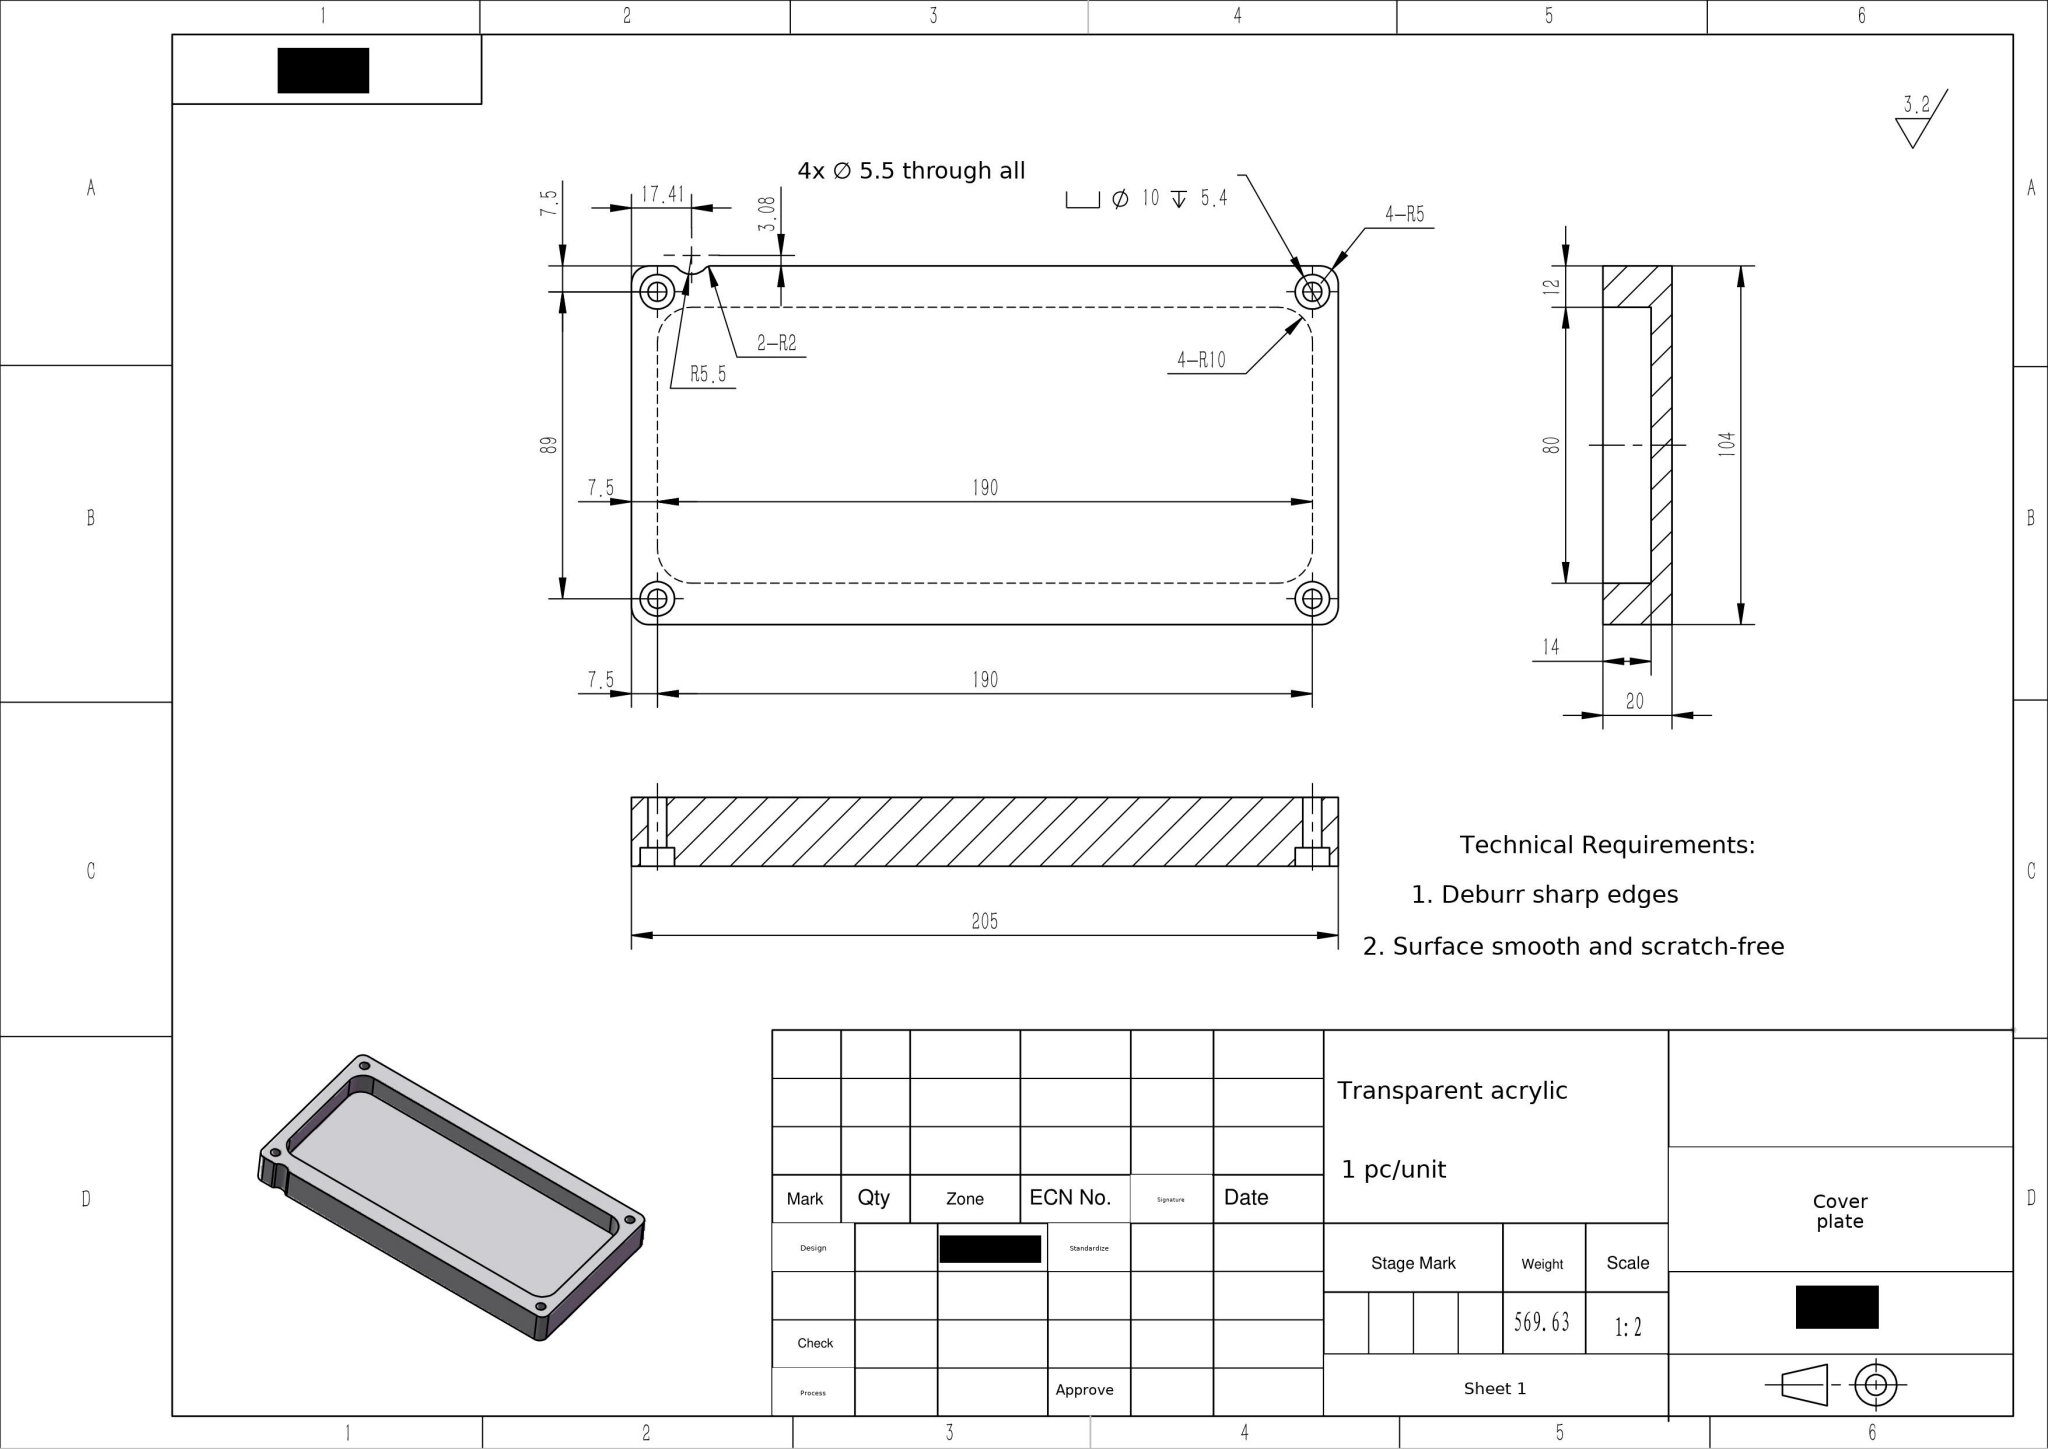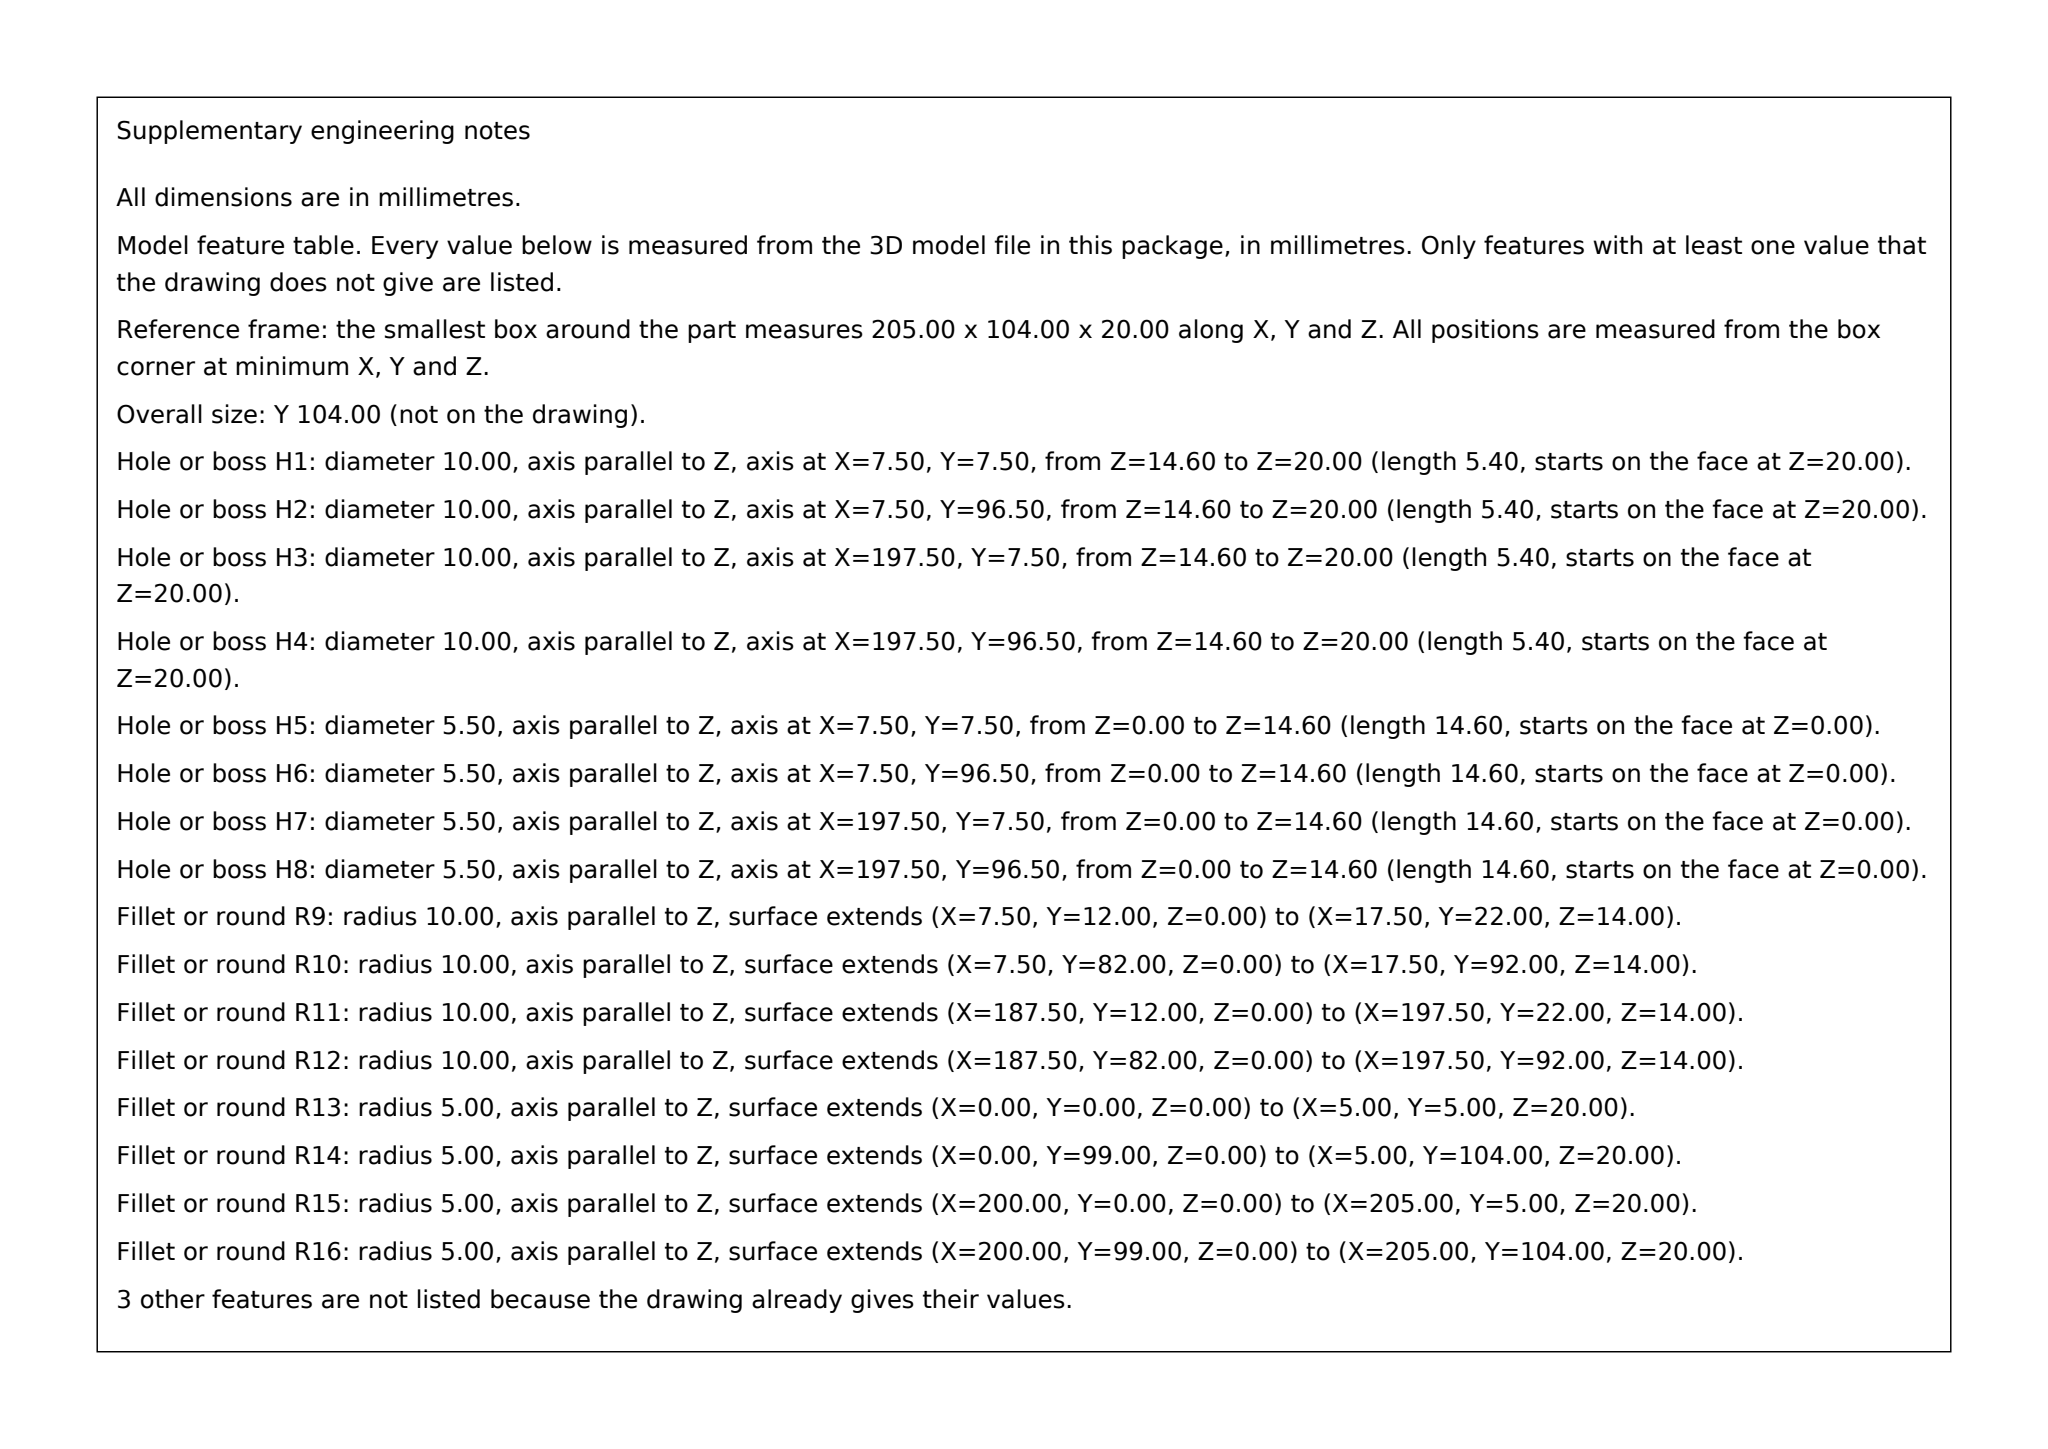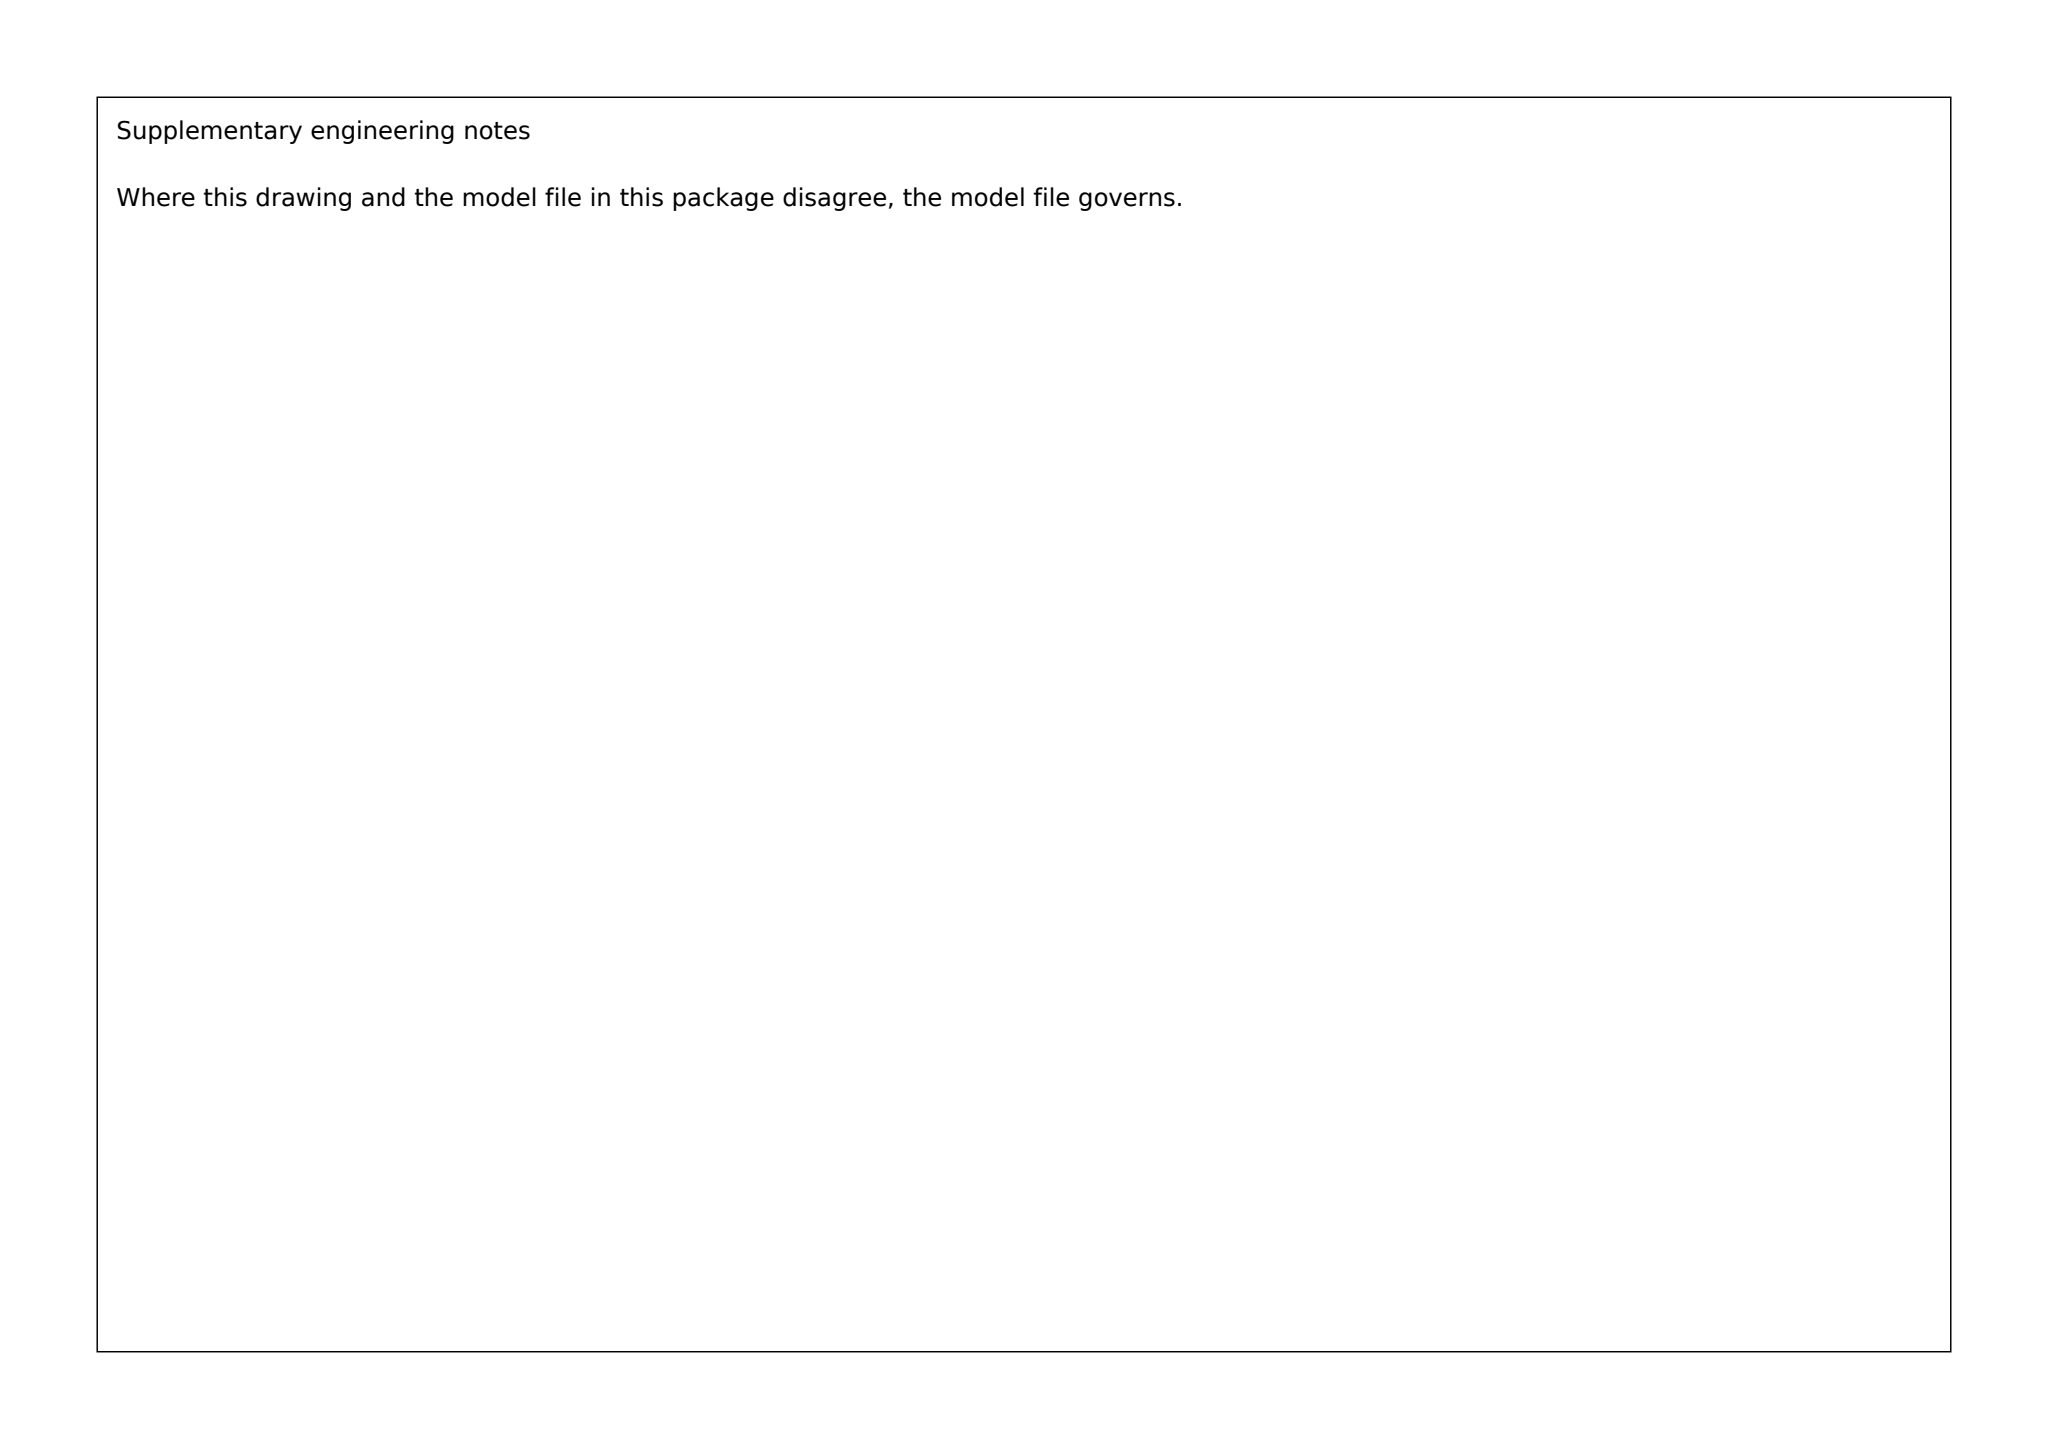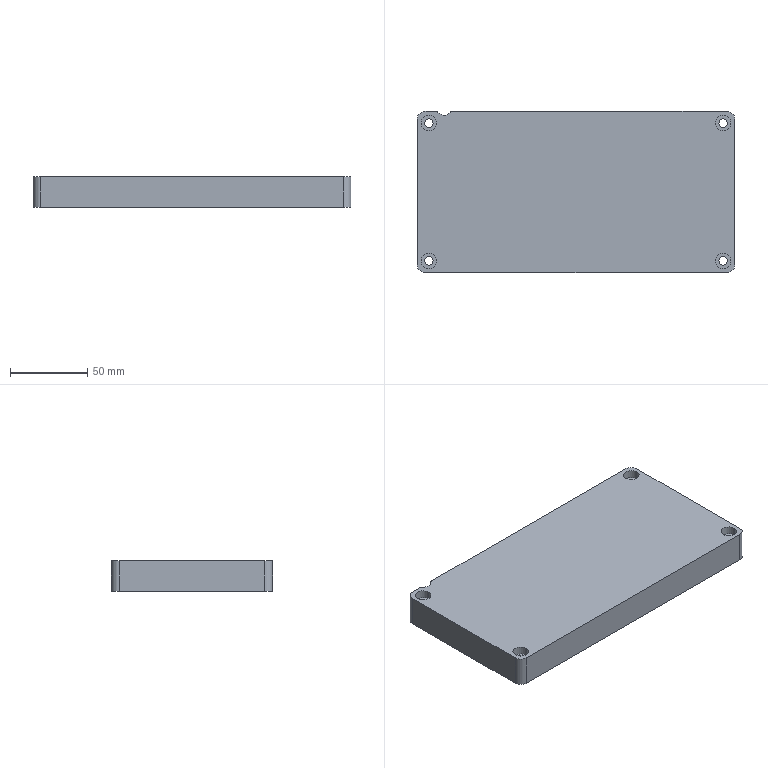Part | SolidWorks | mm | material Transparent acrylic | 1 solid | 43 faces | box 205 x 104 x 20 mm | volume 210974 mm3 | cylinder 27 | plane 16 | commonest cylinder face diameters 10 x12 5.5 x8 20 x4 4 x2 11 x1
build123d program:
from build123d import *

# Parameters (mm, degrees)
SKETCH1_W                                       = 205
SKETCH1_H                                       = 104
BOSS_EXTRUDE1_DEPTH                             = 20
SKETCH2_W                                       = 190
SKETCH2_H                                       = 80
CUT_EXTRUDE1_DEPTH                              = 14
M5_HEX_SOCKET_HEAD_CAP_SCREW_CBORE1_D           = 5.5
M5_HEX_SOCKET_HEAD_CAP_SCREW_CBORE1_CBORE_D     = 10
M5_HEX_SOCKET_HEAD_CAP_SCREW_CBORE1_CBORE_DEPTH = 5.4
FILLET1_R                                       = 10
FILLET2_R                                       = 5
SKETCH5_R                                       = 5.5
CUT_EXTRUDE2_DEPTH                              = 117.663
FILLET3_R                                       = 2


with BuildPart() as part:
    # Sketch1 → Boss-Extrude1 (new body)
    with BuildSketch(Plane.XY):
        Rectangle(SKETCH1_W, SKETCH1_H)
    extrude(amount=BOSS_EXTRUDE1_DEPTH)

    # Sketch2 → Cut-Extrude1 (cut)
    with BuildSketch(Plane.XY):
        Rectangle(SKETCH2_W, SKETCH2_H)
    extrude(amount=CUT_EXTRUDE1_DEPTH, mode=Mode.SUBTRACT)

    # M5 Hex Socket Head Cap Screw CBORE1 (through all)
    with Locations(Plane.XY.offset(20)):
        with Locations((95, -44.5), (-95, -44.5), (95, 44.5), (-95, 44.5)):
            CounterBoreHole(M5_HEX_SOCKET_HEAD_CAP_SCREW_CBORE1_D / 2, M5_HEX_SOCKET_HEAD_CAP_SCREW_CBORE1_CBORE_D / 2, M5_HEX_SOCKET_HEAD_CAP_SCREW_CBORE1_CBORE_DEPTH)

    # Fillet1
    fillet1_edges = [part.edges().sort_by_distance(p)[0] for p in [
        (95, -40, 7),
        (95, 40, 7),
        (-95, 40, 7),
        (-95, -40, 7),
    ]]
    fillet(fillet1_edges, radius=FILLET1_R)

    # Fillet2
    fillet2_edges = [part.edges().sort_by_distance(p)[0] for p in [
        (102.5, -52, 10),
        (-102.5, -52, 10),
        (-102.5, 52, 10),
        (102.5, 52, 10),
    ]]
    fillet(fillet2_edges, radius=FILLET2_R)

    # Sketch5 → Cut-Extrude2 (cut, through all)
    with BuildSketch(Plane.XY.offset(20)):
        with Locations((-85.091, 55.084)):
            Circle(SKETCH5_R)
    extrude(amount=-CUT_EXTRUDE2_DEPTH, mode=Mode.SUBTRACT)

    # Fillet3
    fillet3_edges = [part.edges().sort_by_distance(p)[0] for p in [
        (-80.537, 52, 10),
        (-89.645, 52, 10),
    ]]
    fillet(fillet3_edges, radius=FILLET3_R)


solid = part.part